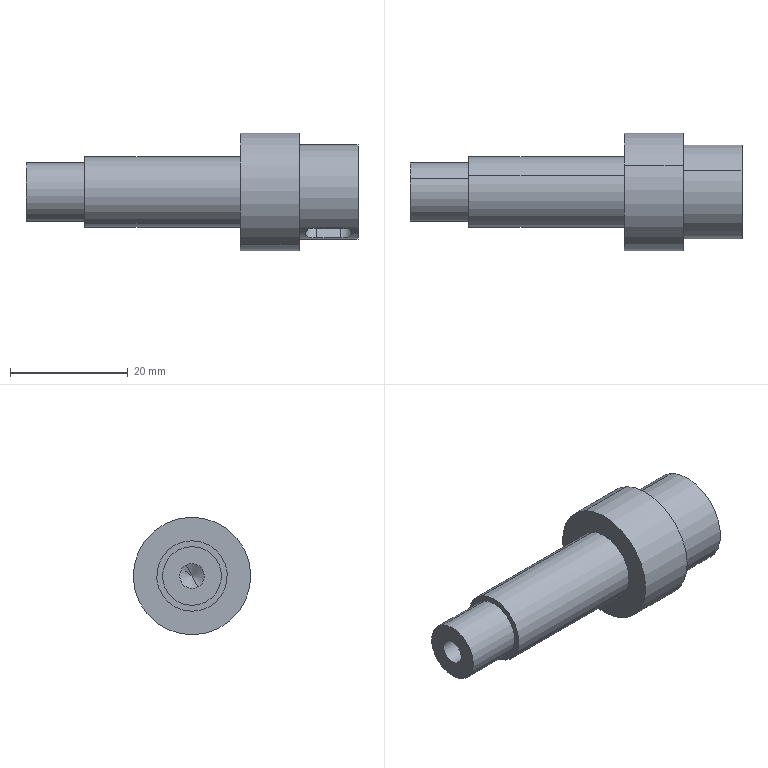Component | SolidWorks | ElectricalBoxAssembly2-1_SwingRodAxis-1 | 1 solid | 27 faces | box 56.5 x 20 x 20 mm | volume 8524 mm3 | cylinder 15 | plane 8 | cone 4 | commonest cylinder face diameters 4.2 x4 4 x3 16 x2 10 x2 12 x2 20 x2
build123d program:
from build123d import *

# Parameters (mm, degrees)
SKETCH1_R             = 10
BOSS_EXTRUDE1_DEPTH   = 10
SKETCH2_R             = 6
BOSS_EXTRUDE2_DEPTH   = 26.5
SKETCH3_R             = 5
BOSS_EXTRUDE3_DEPTH   = 10
M5_TAPPED_HOLE1_D     = 4.2
M5_TAPPED_HOLE1_DEPTH = 12.4
M5_TAPPED_HOLE1_TIP   = 1.262
SKETCH6_R             = 8
BOSS_EXTRUDE4_DEPTH   = 10
CUT_EXTRUDE1_DEPTH    = 2
M5_TAPPED_HOLE2_D     = 4.2
M5_TAPPED_HOLE2_DEPTH = 12.4
M5_TAPPED_HOLE2_TIP   = 1.262


with BuildPart() as part:
    # Sketch1 → Boss-Extrude1 (new body)
    with BuildSketch(Plane.XY):
        Circle(SKETCH1_R)
    extrude(amount=BOSS_EXTRUDE1_DEPTH)

    # Sketch2 → Boss-Extrude2 (add)
    with BuildSketch(Plane.XY.offset(10)):
        Circle(SKETCH2_R)
    extrude(amount=BOSS_EXTRUDE2_DEPTH)

    # Sketch3 → Boss-Extrude3 (add)
    with BuildSketch(Plane.XY.offset(36.5)):
        Circle(SKETCH3_R)
    extrude(amount=BOSS_EXTRUDE3_DEPTH)

    # M5 Tapped Hole1
    with Locations(Plane.XY.offset(46.5)):
        with Locations((0, 0)):
            Hole(M5_TAPPED_HOLE1_D / 2, depth=M5_TAPPED_HOLE1_DEPTH)
            with Locations((0, 0, -(M5_TAPPED_HOLE1_DEPTH + M5_TAPPED_HOLE1_TIP / 2))):  # 118° drill point
                Cone(0, M5_TAPPED_HOLE1_D / 2, M5_TAPPED_HOLE1_TIP, mode=Mode.SUBTRACT)

    # Sketch6 → Boss-Extrude4 (add)
    with BuildSketch(Plane(origin=(0, 0, 0), x_dir=(-1, 0, 0), z_dir=(0, 0, -1))):
        with Locations(Location((0, 0, 0), (0, 0, 180))):
            Circle(SKETCH6_R)
    extrude(amount=BOSS_EXTRUDE4_DEPTH)

    # Sketch7 → Cut-Extrude1 (cut)
    with BuildSketch(Plane(origin=(8, 0, 0), x_dir=(0, 0, -1), z_dir=(1, 0, 0))):
        with BuildLine():
            Line((3, 2), (7, 2))
            ThreePointArc((7, 2), (9, 0), (7, -2))
            Line((7, -2), (3, -2))
            ThreePointArc((3, -2), (1, 0), (3, 2))
        make_face()
    extrude(amount=-CUT_EXTRUDE1_DEPTH, mode=Mode.SUBTRACT)

    # M5 Tapped Hole2
    with Locations(Plane(origin=(0, 0, -10), x_dir=(-1, 0, 0), z_dir=(0, 0, -1))):
        with Locations((0, 0)):
            Hole(M5_TAPPED_HOLE2_D / 2, depth=M5_TAPPED_HOLE2_DEPTH)
            with Locations((0, 0, -(M5_TAPPED_HOLE2_DEPTH + M5_TAPPED_HOLE2_TIP / 2))):  # 118° drill point
                Cone(0, M5_TAPPED_HOLE2_D / 2, M5_TAPPED_HOLE2_TIP, mode=Mode.SUBTRACT)


solid = part.part

# Placed as in the assembly
solid = solid.moved(Location((786.968, 214.666, 1676.399), (152.899, -90, 0)))
STEP:
#1=COLOUR_RGB('',0.7922,0.8196,0.9333);
#2=FILL_AREA_STYLE_COLOUR('',#1);
#3=FILL_AREA_STYLE('',(#2));
#4=SURFACE_STYLE_FILL_AREA(#3);
#5=SURFACE_SIDE_STYLE('',(#4));
#6=SURFACE_STYLE_USAGE(.BOTH.,#5);
#7=PRESENTATION_STYLE_ASSIGNMENT((#6));
#8=CARTESIAN_POINT('',(30.889,8.414,65.926));
#9=VERTEX_POINT('',#8);
#10=CARTESIAN_POINT('',(30.889,8.489,66.074));
#11=VERTEX_POINT('',#10);
#12=CARTESIAN_POINT('',(30.889,8.451,66.));
#13=DIRECTION('',(1.,0.,0.));
#14=DIRECTION('',(0.,0.4556,0.8902));
#15=AXIS2_PLACEMENT_3D('',#12,#13,#14);
#16=CIRCLE('',#15,0.08268);
#17=EDGE_CURVE('',#9,#11,#16,.T.);
#18=ORIENTED_EDGE('',*,*,#17,.F.);
#19=CARTESIAN_POINT('',(31.377,8.414,65.926));
#20=VERTEX_POINT('',#19);
#21=CARTESIAN_POINT('',(31.377,8.414,65.926));
#22=DIRECTION('',(1.,0.,0.));
#23=VECTOR('',#22,39.37);
#24=LINE('',#21,#23);
#25=EDGE_CURVE('',#9,#20,#24,.T.);
#26=ORIENTED_EDGE('',*,*,#25,.T.);
#27=CARTESIAN_POINT('',(31.377,8.489,66.074));
#28=VERTEX_POINT('',#27);
#29=CARTESIAN_POINT('',(31.377,8.451,66.));
#30=DIRECTION('',(1.,0.,0.));
#31=DIRECTION('',(0.,0.4556,0.8902));
#32=AXIS2_PLACEMENT_3D('',#29,#30,#31);
#33=CIRCLE('',#32,0.08268);
#34=EDGE_CURVE('',#20,#28,#33,.T.);
#35=ORIENTED_EDGE('',*,*,#34,.T.);
#36=CARTESIAN_POINT('',(31.377,8.489,66.074));
#37=DIRECTION('',(1.,0.,0.));
#38=VECTOR('',#37,39.37);
#39=LINE('',#36,#38);
#40=EDGE_CURVE('',#11,#28,#39,.T.);
#41=ORIENTED_EDGE('',*,*,#40,.F.);
#42=EDGE_LOOP('',(#18,#26,#35,#41));
#43=FACE_OUTER_BOUND('',#42,.T.);
#44=CARTESIAN_POINT('',(31.377,8.451,66.));
#45=DIRECTION('',(1.,0.,0.));
#46=DIRECTION('',(0.,0.4556,0.8902));
#47=AXIS2_PLACEMENT_3D('',#44,#45,#46);
#48=CYLINDRICAL_SURFACE('',#47,0.08268);
#49=ADVANCED_FACE('',(#43),#48,.F.);
#50=CARTESIAN_POINT('',(30.839,8.451,66.));
#51=VERTEX_POINT('',#50);
#52=CARTESIAN_POINT('',(30.889,8.489,66.074));
#53=DIRECTION('',(0.515,0.3905,0.7631));
#54=VECTOR('',#53,39.37);
#55=LINE('',#52,#54);
#56=EDGE_CURVE('',#51,#11,#55,.T.);
#57=ORIENTED_EDGE('',*,*,#56,.F.);
#58=CARTESIAN_POINT('',(30.889,8.414,65.926));
#59=DIRECTION('',(0.515,-0.3905,-0.7631));
#60=VECTOR('',#59,39.37);
#61=LINE('',#58,#60);
#62=EDGE_CURVE('',#51,#9,#61,.T.);
#63=ORIENTED_EDGE('',*,*,#62,.T.);
#64=ORIENTED_EDGE('',*,*,#17,.T.);
#65=EDGE_LOOP('',(#57,#63,#64));
#66=FACE_OUTER_BOUND('',#65,.T.);
#67=CARTESIAN_POINT('',(30.889,8.451,66.));
#68=DIRECTION('',(1.,0.,0.));
#69=DIRECTION('',(0.,0.4556,0.8902));
#70=AXIS2_PLACEMENT_3D('',#67,#68,#69);
#71=CONICAL_SURFACE('',#70,0.08268,1.03);
#72=ADVANCED_FACE('',(#66),#71,.F.);
#73=CARTESIAN_POINT('',(31.337,8.344,65.79));
#74=VERTEX_POINT('',#73);
#75=CARTESIAN_POINT('',(31.259,8.274,65.826));
#76=VERTEX_POINT('',#75);
#77=CARTESIAN_POINT('',(31.259,8.344,65.79));
#78=DIRECTION('',(0.,-0.4556,-0.8902));
#79=DIRECTION('',(1.,0.,0.));
#80=AXIS2_PLACEMENT_3D('',#77,#78,#79);
#81=CIRCLE('',#80,0.07874);
#82=EDGE_CURVE('',#74,#76,#81,.T.);
#83=ORIENTED_EDGE('',*,*,#82,.F.);
#84=CARTESIAN_POINT('',(31.337,8.308,65.72));
#85=VERTEX_POINT('',#84);
#86=CARTESIAN_POINT('',(31.337,8.344,65.79));
#87=DIRECTION('',(0.,-0.4556,-0.8902));
#88=VECTOR('',#87,39.37);
#89=LINE('',#86,#88);
#90=EDGE_CURVE('',#74,#85,#89,.T.);
#91=ORIENTED_EDGE('',*,*,#90,.T.);
#92=CARTESIAN_POINT('',(31.259,8.242,65.764));
#93=VERTEX_POINT('',#92);
#94=CARTESIAN_POINT('',(31.259,8.242,65.764));
#95=CARTESIAN_POINT('',(31.264,8.242,65.764));
#96=CARTESIAN_POINT('',(31.269,8.243,65.764));
#97=CARTESIAN_POINT('',(31.279,8.244,65.763));
#98=CARTESIAN_POINT('',(31.284,8.246,65.762));
#99=CARTESIAN_POINT('',(31.294,8.249,65.759));
#100=CARTESIAN_POINT('',(31.298,8.251,65.757));
#101=CARTESIAN_POINT('',(31.307,8.255,65.754));
#102=CARTESIAN_POINT('',(31.311,8.258,65.752));
#103=CARTESIAN_POINT('',(31.322,8.266,65.745));
#104=CARTESIAN_POINT('',(31.327,8.274,65.74));
#105=CARTESIAN_POINT('',(31.333,8.286,65.732));
#106=CARTESIAN_POINT('',(31.335,8.29,65.729));
#107=CARTESIAN_POINT('',(31.337,8.299,65.724));
#108=CARTESIAN_POINT('',(31.337,8.303,65.722));
#109=CARTESIAN_POINT('',(31.337,8.308,65.72));
#110=B_SPLINE_CURVE_WITH_KNOTS('',3,(#94,#95,#96,#97,#98,#99,#100,#101,#102,#103,#104,#105,#106,#107,#108,#109),.UNSPECIFIED.,.F.,.F.,(4,2,2,2,2,2,2,4),(0.,0.0003925,0.0007849,0.001177,0.00157,0.002355,0.002747,0.00314),.UNSPECIFIED.);
#111=EDGE_CURVE('',#93,#85,#110,.T.);
#112=ORIENTED_EDGE('',*,*,#111,.F.);
#113=CARTESIAN_POINT('',(31.259,8.274,65.826));
#114=DIRECTION('',(0.,-0.4556,-0.8902));
#115=VECTOR('',#114,39.37);
#116=LINE('',#113,#115);
#117=EDGE_CURVE('',#76,#93,#116,.T.);
#118=ORIENTED_EDGE('',*,*,#117,.F.);
#119=EDGE_LOOP('',(#83,#91,#112,#118));
#120=FACE_OUTER_BOUND('',#119,.T.);
#121=CARTESIAN_POINT('',(31.259,8.344,65.79));
#122=DIRECTION('',(0.,-0.4556,-0.8902));
#123=DIRECTION('',(1.,0.,0.));
#124=AXIS2_PLACEMENT_3D('',#121,#122,#123);
#125=CYLINDRICAL_SURFACE('',#124,0.07874);
#126=ADVANCED_FACE('',(#120),#125,.F.);
#127=CARTESIAN_POINT('',(31.377,8.595,66.28));
#128=VERTEX_POINT('',#127);
#129=CARTESIAN_POINT('',(31.377,8.308,65.72));
#130=VERTEX_POINT('',#129);
#131=CARTESIAN_POINT('',(31.377,8.451,66.));
#132=DIRECTION('',(1.,0.,0.));
#133=DIRECTION('',(0.,0.4556,0.8902));
#134=AXIS2_PLACEMENT_3D('',#131,#132,#133);
#135=CIRCLE('',#134,0.315);
#136=EDGE_CURVE('',#128,#130,#135,.T.);
#137=ORIENTED_EDGE('',*,*,#136,.F.);
#138=CARTESIAN_POINT('',(30.983,8.595,66.28));
#139=VERTEX_POINT('',#138);
#140=CARTESIAN_POINT('',(31.377,8.595,66.28));
#141=DIRECTION('',(-1.,-0.,-0.));
#142=VECTOR('',#141,39.37);
#143=LINE('',#140,#142);
#144=EDGE_CURVE('',#128,#139,#143,.T.);
#145=ORIENTED_EDGE('',*,*,#144,.T.);
#146=CARTESIAN_POINT('',(30.983,8.308,65.72));
#147=VERTEX_POINT('',#146);
#148=CARTESIAN_POINT('',(30.983,8.451,66.));
#149=DIRECTION('',(1.,0.,0.));
#150=DIRECTION('',(0.,-0.4556,-0.8902));
#151=AXIS2_PLACEMENT_3D('',#148,#149,#150);
#152=CIRCLE('',#151,0.315);
#153=EDGE_CURVE('',#139,#147,#152,.T.);
#154=ORIENTED_EDGE('',*,*,#153,.T.);
#155=CARTESIAN_POINT('',(31.022,8.308,65.72));
#156=VERTEX_POINT('',#155);
#157=CARTESIAN_POINT('',(31.377,8.308,65.72));
#158=DIRECTION('',(-1.,-0.,-0.));
#159=VECTOR('',#158,39.37);
#160=LINE('',#157,#159);
#161=EDGE_CURVE('',#156,#147,#160,.T.);
#162=ORIENTED_EDGE('',*,*,#161,.F.);
#163=CARTESIAN_POINT('',(31.101,8.242,65.764));
#164=VERTEX_POINT('',#163);
#165=CARTESIAN_POINT('',(31.022,8.308,65.72));
#166=CARTESIAN_POINT('',(31.022,8.303,65.722));
#167=CARTESIAN_POINT('',(31.023,8.299,65.724));
#168=CARTESIAN_POINT('',(31.025,8.29,65.729));
#169=CARTESIAN_POINT('',(31.026,8.286,65.732));
#170=CARTESIAN_POINT('',(31.032,8.274,65.74));
#171=CARTESIAN_POINT('',(31.038,8.267,65.745));
#172=CARTESIAN_POINT('',(31.049,8.258,65.752));
#173=CARTESIAN_POINT('',(31.053,8.255,65.754));
#174=CARTESIAN_POINT('',(31.062,8.251,65.757));
#175=CARTESIAN_POINT('',(31.066,8.249,65.759));
#176=CARTESIAN_POINT('',(31.076,8.246,65.762));
#177=CARTESIAN_POINT('',(31.081,8.244,65.763));
#178=CARTESIAN_POINT('',(31.091,8.243,65.764));
#179=CARTESIAN_POINT('',(31.096,8.242,65.764));
#180=CARTESIAN_POINT('',(31.101,8.242,65.764));
#181=B_SPLINE_CURVE_WITH_KNOTS('',3,(#165,#166,#167,#168,#169,#170,#171,#172,#173,#174,#175,#176,#177,#178,#179,#180),.UNSPECIFIED.,.F.,.F.,(4,2,2,2,2,2,2,4),(0.00314,0.003532,0.003924,0.004708,0.0051,0.005492,0.005884,0.006276),.UNSPECIFIED.);
#182=EDGE_CURVE('',#156,#164,#181,.T.);
#183=ORIENTED_EDGE('',*,*,#182,.T.);
#184=CARTESIAN_POINT('',(31.377,8.242,65.764));
#185=DIRECTION('',(1.,0.,0.));
#186=VECTOR('',#185,39.37);
#187=LINE('',#184,#186);
#188=EDGE_CURVE('',#164,#93,#187,.T.);
#189=ORIENTED_EDGE('',*,*,#188,.T.);
#190=ORIENTED_EDGE('',*,*,#111,.T.);
#191=CARTESIAN_POINT('',(31.377,8.308,65.72));
#192=DIRECTION('',(-1.,-0.,-0.));
#193=VECTOR('',#192,39.37);
#194=LINE('',#191,#193);
#195=EDGE_CURVE('',#130,#85,#194,.T.);
#196=ORIENTED_EDGE('',*,*,#195,.F.);
#197=EDGE_LOOP('',(#137,#145,#154,#162,#183,#189,#190,#196));
#198=FACE_OUTER_BOUND('',#197,.T.);
#199=CARTESIAN_POINT('',(31.377,8.451,66.));
#200=DIRECTION('',(-1.,-0.,-0.));
#201=DIRECTION('',(0.,-0.4556,-0.8902));
#202=AXIS2_PLACEMENT_3D('',#199,#200,#201);
#203=CYLINDRICAL_SURFACE('',#202,0.315);
#204=ADVANCED_FACE('',(#198),#203,.T.);
#205=CARTESIAN_POINT('',(29.64,8.489,66.074));
#206=VERTEX_POINT('',#205);
#207=CARTESIAN_POINT('',(29.64,8.414,65.926));
#208=VERTEX_POINT('',#207);
#209=CARTESIAN_POINT('',(29.64,8.451,66.));
#210=DIRECTION('',(-1.,-0.,-0.));
#211=DIRECTION('',(0.,-0.4556,-0.8902));
#212=AXIS2_PLACEMENT_3D('',#209,#210,#211);
#213=CIRCLE('',#212,0.08268);
#214=EDGE_CURVE('',#206,#208,#213,.T.);
#215=ORIENTED_EDGE('',*,*,#214,.F.);
#216=CARTESIAN_POINT('',(29.152,8.489,66.074));
#217=VERTEX_POINT('',#216);
#218=CARTESIAN_POINT('',(29.152,8.489,66.074));
#219=DIRECTION('',(-1.,-0.,-0.));
#220=VECTOR('',#219,39.37);
#221=LINE('',#218,#220);
#222=EDGE_CURVE('',#206,#217,#221,.T.);
#223=ORIENTED_EDGE('',*,*,#222,.T.);
#224=CARTESIAN_POINT('',(29.152,8.414,65.926));
#225=VERTEX_POINT('',#224);
#226=CARTESIAN_POINT('',(29.152,8.451,66.));
#227=DIRECTION('',(-1.,-0.,-0.));
#228=DIRECTION('',(0.,-0.4556,-0.8902));
#229=AXIS2_PLACEMENT_3D('',#226,#227,#228);
#230=CIRCLE('',#229,0.08268);
#231=EDGE_CURVE('',#217,#225,#230,.T.);
#232=ORIENTED_EDGE('',*,*,#231,.T.);
#233=CARTESIAN_POINT('',(29.152,8.414,65.926));
#234=DIRECTION('',(-1.,-0.,-0.));
#235=VECTOR('',#234,39.37);
#236=LINE('',#233,#235);
#237=EDGE_CURVE('',#208,#225,#236,.T.);
#238=ORIENTED_EDGE('',*,*,#237,.F.);
#239=EDGE_LOOP('',(#215,#223,#232,#238));
#240=FACE_OUTER_BOUND('',#239,.T.);
#241=CARTESIAN_POINT('',(29.152,8.451,66.));
#242=DIRECTION('',(-1.,-0.,-0.));
#243=DIRECTION('',(0.,-0.4556,-0.8902));
#244=AXIS2_PLACEMENT_3D('',#241,#242,#243);
#245=CYLINDRICAL_SURFACE('',#244,0.08268);
#246=ADVANCED_FACE('',(#240),#245,.F.);
#247=CARTESIAN_POINT('',(29.69,8.451,66.));
#248=VERTEX_POINT('',#247);
#249=CARTESIAN_POINT('',(29.64,8.414,65.926));
#250=DIRECTION('',(-0.515,-0.3905,-0.7631));
#251=VECTOR('',#250,39.37);
#252=LINE('',#249,#251);
#253=EDGE_CURVE('',#248,#208,#252,.T.);
#254=ORIENTED_EDGE('',*,*,#253,.F.);
#255=CARTESIAN_POINT('',(29.64,8.489,66.074));
#256=DIRECTION('',(-0.515,0.3905,0.7631));
#257=VECTOR('',#256,39.37);
#258=LINE('',#255,#257);
#259=EDGE_CURVE('',#248,#206,#258,.T.);
#260=ORIENTED_EDGE('',*,*,#259,.T.);
#261=ORIENTED_EDGE('',*,*,#214,.T.);
#262=EDGE_LOOP('',(#254,#260,#261));
#263=FACE_OUTER_BOUND('',#262,.T.);
#264=CARTESIAN_POINT('',(29.64,8.451,66.));
#265=DIRECTION('',(-1.,-0.,-0.));
#266=DIRECTION('',(0.,-0.4556,-0.8902));
#267=AXIS2_PLACEMENT_3D('',#264,#265,#266);
#268=CONICAL_SURFACE('',#267,0.08268,1.03);
#269=ADVANCED_FACE('',(#263),#268,.F.);
#270=CARTESIAN_POINT('',(29.152,8.362,65.825));
#271=VERTEX_POINT('',#270);
#272=CARTESIAN_POINT('',(29.152,8.541,66.175));
#273=VERTEX_POINT('',#272);
#274=CARTESIAN_POINT('',(29.152,8.451,66.));
#275=DIRECTION('',(-1.,-0.,-0.));
#276=DIRECTION('',(0.,-0.4556,-0.8902));
#277=AXIS2_PLACEMENT_3D('',#274,#275,#276);
#278=CIRCLE('',#277,0.1969);
#279=EDGE_CURVE('',#271,#273,#278,.T.);
#280=ORIENTED_EDGE('',*,*,#279,.F.);
#281=CARTESIAN_POINT('',(29.546,8.362,65.825));
#282=VERTEX_POINT('',#281);
#283=CARTESIAN_POINT('',(29.152,8.362,65.825));
#284=DIRECTION('',(1.,0.,0.));
#285=VECTOR('',#284,39.37);
#286=LINE('',#283,#285);
#287=EDGE_CURVE('',#271,#282,#286,.T.);
#288=ORIENTED_EDGE('',*,*,#287,.T.);
#289=CARTESIAN_POINT('',(29.546,8.541,66.175));
#290=VERTEX_POINT('',#289);
#291=CARTESIAN_POINT('',(29.546,8.451,66.));
#292=DIRECTION('',(-1.,-0.,-0.));
#293=DIRECTION('',(0.,-0.4556,-0.8902));
#294=AXIS2_PLACEMENT_3D('',#291,#292,#293);
#295=CIRCLE('',#294,0.1969);
#296=EDGE_CURVE('',#282,#290,#295,.T.);
#297=ORIENTED_EDGE('',*,*,#296,.T.);
#298=CARTESIAN_POINT('',(29.152,8.541,66.175));
#299=DIRECTION('',(1.,0.,0.));
#300=VECTOR('',#299,39.37);
#301=LINE('',#298,#300);
#302=EDGE_CURVE('',#273,#290,#301,.T.);
#303=ORIENTED_EDGE('',*,*,#302,.F.);
#304=EDGE_LOOP('',(#280,#288,#297,#303));
#305=FACE_OUTER_BOUND('',#304,.T.);
#306=CARTESIAN_POINT('',(29.152,8.451,66.));
#307=DIRECTION('',(1.,0.,0.));
#308=DIRECTION('',(0.,0.4556,0.8902));
#309=AXIS2_PLACEMENT_3D('',#306,#307,#308);
#310=CYLINDRICAL_SURFACE('',#309,0.1969);
#311=ADVANCED_FACE('',(#305),#310,.T.);
#312=CARTESIAN_POINT('',(29.546,8.344,65.79));
#313=VERTEX_POINT('',#312);
#314=CARTESIAN_POINT('',(29.546,8.559,66.21));
#315=VERTEX_POINT('',#314);
#316=CARTESIAN_POINT('',(29.546,8.451,66.));
#317=DIRECTION('',(-1.,-0.,-0.));
#318=DIRECTION('',(0.,-0.4556,-0.8902));
#319=AXIS2_PLACEMENT_3D('',#316,#317,#318);
#320=CIRCLE('',#319,0.2362);
#321=EDGE_CURVE('',#313,#315,#320,.T.);
#322=ORIENTED_EDGE('',*,*,#321,.F.);
#323=CARTESIAN_POINT('',(30.589,8.344,65.79));
#324=VERTEX_POINT('',#323);
#325=CARTESIAN_POINT('',(29.546,8.344,65.79));
#326=DIRECTION('',(1.,0.,0.));
#327=VECTOR('',#326,39.37);
#328=LINE('',#325,#327);
#329=EDGE_CURVE('',#313,#324,#328,.T.);
#330=ORIENTED_EDGE('',*,*,#329,.T.);
#331=CARTESIAN_POINT('',(30.589,8.559,66.21));
#332=VERTEX_POINT('',#331);
#333=CARTESIAN_POINT('',(30.589,8.451,66.));
#334=DIRECTION('',(-1.,-0.,-0.));
#335=DIRECTION('',(0.,-0.4556,-0.8902));
#336=AXIS2_PLACEMENT_3D('',#333,#334,#335);
#337=CIRCLE('',#336,0.2362);
#338=EDGE_CURVE('',#324,#332,#337,.T.);
#339=ORIENTED_EDGE('',*,*,#338,.T.);
#340=CARTESIAN_POINT('',(29.546,8.559,66.21));
#341=DIRECTION('',(1.,0.,0.));
#342=VECTOR('',#341,39.37);
#343=LINE('',#340,#342);
#344=EDGE_CURVE('',#315,#332,#343,.T.);
#345=ORIENTED_EDGE('',*,*,#344,.F.);
#346=EDGE_LOOP('',(#322,#330,#339,#345));
#347=FACE_OUTER_BOUND('',#346,.T.);
#348=CARTESIAN_POINT('',(29.546,8.451,66.));
#349=DIRECTION('',(1.,0.,0.));
#350=DIRECTION('',(0.,0.4556,0.8902));
#351=AXIS2_PLACEMENT_3D('',#348,#349,#350);
#352=CYLINDRICAL_SURFACE('',#351,0.2362);
#353=ADVANCED_FACE('',(#347),#352,.T.);
#354=CARTESIAN_POINT('',(30.589,8.272,65.649));
#355=VERTEX_POINT('',#354);
#356=CARTESIAN_POINT('',(30.589,8.631,66.35));
#357=VERTEX_POINT('',#356);
#358=CARTESIAN_POINT('',(30.589,8.451,66.));
#359=DIRECTION('',(-1.,-0.,-0.));
#360=DIRECTION('',(0.,-0.4556,-0.8902));
#361=AXIS2_PLACEMENT_3D('',#358,#359,#360);
#362=CIRCLE('',#361,0.3937);
#363=EDGE_CURVE('',#355,#357,#362,.T.);
#364=ORIENTED_EDGE('',*,*,#363,.F.);
#365=CARTESIAN_POINT('',(30.983,8.272,65.649));
#366=VERTEX_POINT('',#365);
#367=CARTESIAN_POINT('',(30.589,8.272,65.649));
#368=DIRECTION('',(1.,0.,0.));
#369=VECTOR('',#368,39.37);
#370=LINE('',#367,#369);
#371=EDGE_CURVE('',#355,#366,#370,.T.);
#372=ORIENTED_EDGE('',*,*,#371,.T.);
#373=CARTESIAN_POINT('',(30.983,8.631,66.35));
#374=VERTEX_POINT('',#373);
#375=CARTESIAN_POINT('',(30.983,8.451,66.));
#376=DIRECTION('',(-1.,-0.,-0.));
#377=DIRECTION('',(0.,-0.4556,-0.8902));
#378=AXIS2_PLACEMENT_3D('',#375,#376,#377);
#379=CIRCLE('',#378,0.3937);
#380=EDGE_CURVE('',#366,#374,#379,.T.);
#381=ORIENTED_EDGE('',*,*,#380,.T.);
#382=CARTESIAN_POINT('',(30.589,8.631,66.35));
#383=DIRECTION('',(1.,0.,0.));
#384=VECTOR('',#383,39.37);
#385=LINE('',#382,#384);
#386=EDGE_CURVE('',#357,#374,#385,.T.);
#387=ORIENTED_EDGE('',*,*,#386,.F.);
#388=EDGE_LOOP('',(#364,#372,#381,#387));
#389=FACE_OUTER_BOUND('',#388,.T.);
#390=CARTESIAN_POINT('',(30.589,8.451,66.));
#391=DIRECTION('',(1.,0.,0.));
#392=DIRECTION('',(0.,0.4556,0.8902));
#393=AXIS2_PLACEMENT_3D('',#390,#391,#392);
#394=CYLINDRICAL_SURFACE('',#393,0.3937);
#395=ADVANCED_FACE('',(#389),#394,.T.);
#396=ORIENTED_EDGE('',*,*,#371,.F.);
#397=CARTESIAN_POINT('',(30.589,8.451,66.));
#398=DIRECTION('',(-1.,-0.,-0.));
#399=DIRECTION('',(0.,-0.4556,-0.8902));
#400=AXIS2_PLACEMENT_3D('',#397,#398,#399);
#401=CIRCLE('',#400,0.3937);
#402=EDGE_CURVE('',#357,#355,#401,.T.);
#403=ORIENTED_EDGE('',*,*,#402,.F.);
#404=ORIENTED_EDGE('',*,*,#386,.T.);
#405=CARTESIAN_POINT('',(30.983,8.451,66.));
#406=DIRECTION('',(-1.,-0.,-0.));
#407=DIRECTION('',(0.,-0.4556,-0.8902));
#408=AXIS2_PLACEMENT_3D('',#405,#406,#407);
#409=CIRCLE('',#408,0.3937);
#410=EDGE_CURVE('',#374,#366,#409,.T.);
#411=ORIENTED_EDGE('',*,*,#410,.T.);
#412=EDGE_LOOP('',(#396,#403,#404,#411));
#413=FACE_OUTER_BOUND('',#412,.T.);
#414=CARTESIAN_POINT('',(30.589,8.451,66.));
#415=DIRECTION('',(1.,0.,0.));
#416=DIRECTION('',(0.,0.4556,0.8902));
#417=AXIS2_PLACEMENT_3D('',#414,#415,#416);
#418=CYLINDRICAL_SURFACE('',#417,0.3937);
#419=ADVANCED_FACE('',(#413),#418,.T.);
#420=CARTESIAN_POINT('',(30.589,8.451,66.));
#421=DIRECTION('',(-1.,-0.,-0.));
#422=DIRECTION('',(0.,-0.4556,-0.8902));
#423=AXIS2_PLACEMENT_3D('',#420,#421,#422);
#424=CIRCLE('',#423,0.2362);
#425=EDGE_CURVE('',#332,#324,#424,.T.);
#426=ORIENTED_EDGE('',*,*,#425,.F.);
#427=ORIENTED_EDGE('',*,*,#338,.F.);
#428=EDGE_LOOP('',(#426,#427));
#429=FACE_BOUND('',#428,.T.);
#430=ORIENTED_EDGE('',*,*,#402,.T.);
#431=ORIENTED_EDGE('',*,*,#363,.T.);
#432=EDGE_LOOP('',(#430,#431));
#433=FACE_OUTER_BOUND('',#432,.T.);
#434=CARTESIAN_POINT('',(30.589,8.451,66.));
#435=DIRECTION('',(-1.,-0.,-0.));
#436=DIRECTION('',(0.,-0.4556,-0.8902));
#437=AXIS2_PLACEMENT_3D('',#434,#435,#436);
#438=PLANE('',#437);
#439=ADVANCED_FACE('',(#429,#433),#438,.T.);
#440=CARTESIAN_POINT('',(30.983,8.451,66.));
#441=DIRECTION('',(1.,0.,0.));
#442=DIRECTION('',(0.,-0.4556,-0.8902));
#443=AXIS2_PLACEMENT_3D('',#440,#441,#442);
#444=CIRCLE('',#443,0.315);
#445=EDGE_CURVE('',#147,#139,#444,.T.);
#446=ORIENTED_EDGE('',*,*,#445,.F.);
#447=ORIENTED_EDGE('',*,*,#153,.F.);
#448=EDGE_LOOP('',(#446,#447));
#449=FACE_BOUND('',#448,.T.);
#450=ORIENTED_EDGE('',*,*,#410,.F.);
#451=ORIENTED_EDGE('',*,*,#380,.F.);
#452=EDGE_LOOP('',(#450,#451));
#453=FACE_OUTER_BOUND('',#452,.T.);
#454=CARTESIAN_POINT('',(30.983,8.451,66.));
#455=DIRECTION('',(-1.,-0.,-0.));
#456=DIRECTION('',(0.,-0.4556,-0.8902));
#457=AXIS2_PLACEMENT_3D('',#454,#455,#456);
#458=PLANE('',#457);
#459=ADVANCED_FACE('',(#449,#453),#458,.F.);
#460=ORIENTED_EDGE('',*,*,#329,.F.);
#461=CARTESIAN_POINT('',(29.546,8.451,66.));
#462=DIRECTION('',(-1.,-0.,-0.));
#463=DIRECTION('',(0.,-0.4556,-0.8902));
#464=AXIS2_PLACEMENT_3D('',#461,#462,#463);
#465=CIRCLE('',#464,0.2362);
#466=EDGE_CURVE('',#315,#313,#465,.T.);
#467=ORIENTED_EDGE('',*,*,#466,.F.);
#468=ORIENTED_EDGE('',*,*,#344,.T.);
#469=ORIENTED_EDGE('',*,*,#425,.T.);
#470=EDGE_LOOP('',(#460,#467,#468,#469));
#471=FACE_OUTER_BOUND('',#470,.T.);
#472=CARTESIAN_POINT('',(29.546,8.451,66.));
#473=DIRECTION('',(1.,0.,0.));
#474=DIRECTION('',(0.,0.4556,0.8902));
#475=AXIS2_PLACEMENT_3D('',#472,#473,#474);
#476=CYLINDRICAL_SURFACE('',#475,0.2362);
#477=ADVANCED_FACE('',(#471),#476,.T.);
#478=CARTESIAN_POINT('',(29.546,8.451,66.));
#479=DIRECTION('',(-1.,-0.,-0.));
#480=DIRECTION('',(0.,-0.4556,-0.8902));
#481=AXIS2_PLACEMENT_3D('',#478,#479,#480);
#482=CIRCLE('',#481,0.1969);
#483=EDGE_CURVE('',#290,#282,#482,.T.);
#484=ORIENTED_EDGE('',*,*,#483,.F.);
#485=ORIENTED_EDGE('',*,*,#296,.F.);
#486=EDGE_LOOP('',(#484,#485));
#487=FACE_BOUND('',#486,.T.);
#488=ORIENTED_EDGE('',*,*,#466,.T.);
#489=ORIENTED_EDGE('',*,*,#321,.T.);
#490=EDGE_LOOP('',(#488,#489));
#491=FACE_OUTER_BOUND('',#490,.T.);
#492=CARTESIAN_POINT('',(29.546,8.451,66.));
#493=DIRECTION('',(-1.,-0.,-0.));
#494=DIRECTION('',(0.,-0.4556,-0.8902));
#495=AXIS2_PLACEMENT_3D('',#492,#493,#494);
#496=PLANE('',#495);
#497=ADVANCED_FACE('',(#487,#491),#496,.T.);
#498=ORIENTED_EDGE('',*,*,#287,.F.);
#499=CARTESIAN_POINT('',(29.152,8.451,66.));
#500=DIRECTION('',(-1.,-0.,-0.));
#501=DIRECTION('',(0.,-0.4556,-0.8902));
#502=AXIS2_PLACEMENT_3D('',#499,#500,#501);
#503=CIRCLE('',#502,0.1969);
#504=EDGE_CURVE('',#273,#271,#503,.T.);
#505=ORIENTED_EDGE('',*,*,#504,.F.);
#506=ORIENTED_EDGE('',*,*,#302,.T.);
#507=ORIENTED_EDGE('',*,*,#483,.T.);
#508=EDGE_LOOP('',(#498,#505,#506,#507));
#509=FACE_OUTER_BOUND('',#508,.T.);
#510=CARTESIAN_POINT('',(29.152,8.451,66.));
#511=DIRECTION('',(1.,0.,0.));
#512=DIRECTION('',(0.,0.4556,0.8902));
#513=AXIS2_PLACEMENT_3D('',#510,#511,#512);
#514=CYLINDRICAL_SURFACE('',#513,0.1969);
#515=ADVANCED_FACE('',(#509),#514,.T.);
#516=CARTESIAN_POINT('',(29.152,8.451,66.));
#517=DIRECTION('',(-1.,-0.,-0.));
#518=DIRECTION('',(0.,-0.4556,-0.8902));
#519=AXIS2_PLACEMENT_3D('',#516,#517,#518);
#520=CIRCLE('',#519,0.08268);
#521=EDGE_CURVE('',#225,#217,#520,.T.);
#522=ORIENTED_EDGE('',*,*,#521,.F.);
#523=ORIENTED_EDGE('',*,*,#231,.F.);
#524=EDGE_LOOP('',(#522,#523));
#525=FACE_BOUND('',#524,.T.);
#526=ORIENTED_EDGE('',*,*,#504,.T.);
#527=ORIENTED_EDGE('',*,*,#279,.T.);
#528=EDGE_LOOP('',(#526,#527));
#529=FACE_OUTER_BOUND('',#528,.T.);
#530=CARTESIAN_POINT('',(29.152,8.451,66.));
#531=DIRECTION('',(-1.,-0.,-0.));
#532=DIRECTION('',(0.,-0.4556,-0.8902));
#533=AXIS2_PLACEMENT_3D('',#530,#531,#532);
#534=PLANE('',#533);
#535=ADVANCED_FACE('',(#525,#529),#534,.T.);
#536=ORIENTED_EDGE('',*,*,#259,.F.);
#537=ORIENTED_EDGE('',*,*,#253,.T.);
#538=CARTESIAN_POINT('',(29.64,8.451,66.));
#539=DIRECTION('',(-1.,-0.,-0.));
#540=DIRECTION('',(0.,-0.4556,-0.8902));
#541=AXIS2_PLACEMENT_3D('',#538,#539,#540);
#542=CIRCLE('',#541,0.08268);
#543=EDGE_CURVE('',#208,#206,#542,.T.);
#544=ORIENTED_EDGE('',*,*,#543,.T.);
#545=EDGE_LOOP('',(#536,#537,#544));
#546=FACE_OUTER_BOUND('',#545,.T.);
#547=CARTESIAN_POINT('',(29.64,8.451,66.));
#548=DIRECTION('',(-1.,-0.,-0.));
#549=DIRECTION('',(0.,-0.4556,-0.8902));
#550=AXIS2_PLACEMENT_3D('',#547,#548,#549);
#551=CONICAL_SURFACE('',#550,0.08268,1.03);
#552=ADVANCED_FACE('',(#546),#551,.F.);
#553=ORIENTED_EDGE('',*,*,#222,.F.);
#554=ORIENTED_EDGE('',*,*,#543,.F.);
#555=ORIENTED_EDGE('',*,*,#237,.T.);
#556=ORIENTED_EDGE('',*,*,#521,.T.);
#557=EDGE_LOOP('',(#553,#554,#555,#556));
#558=FACE_OUTER_BOUND('',#557,.T.);
#559=CARTESIAN_POINT('',(29.152,8.451,66.));
#560=DIRECTION('',(-1.,-0.,-0.));
#561=DIRECTION('',(0.,-0.4556,-0.8902));
#562=AXIS2_PLACEMENT_3D('',#559,#560,#561);
#563=CYLINDRICAL_SURFACE('',#562,0.08268);
#564=ADVANCED_FACE('',(#558),#563,.F.);
#565=ORIENTED_EDGE('',*,*,#144,.F.);
#566=CARTESIAN_POINT('',(31.377,8.451,66.));
#567=DIRECTION('',(1.,0.,0.));
#568=DIRECTION('',(0.,0.4556,0.8902));
#569=AXIS2_PLACEMENT_3D('',#566,#567,#568);
#570=CIRCLE('',#569,0.315);
#571=EDGE_CURVE('',#130,#128,#570,.T.);
#572=ORIENTED_EDGE('',*,*,#571,.F.);
#573=ORIENTED_EDGE('',*,*,#195,.T.);
#574=CARTESIAN_POINT('',(31.259,8.383,65.693));
#575=VERTEX_POINT('',#574);
#576=CARTESIAN_POINT('',(31.337,8.308,65.72));
#577=CARTESIAN_POINT('',(31.337,8.313,65.717));
#578=CARTESIAN_POINT('',(31.337,8.317,65.715));
#579=CARTESIAN_POINT('',(31.335,8.326,65.711));
#580=CARTESIAN_POINT('',(31.333,8.331,65.709));
#581=CARTESIAN_POINT('',(31.327,8.344,65.704));
#582=CARTESIAN_POINT('',(31.322,8.353,65.701));
#583=CARTESIAN_POINT('',(31.311,8.363,65.698));
#584=CARTESIAN_POINT('',(31.307,8.366,65.697));
#585=CARTESIAN_POINT('',(31.298,8.372,65.695));
#586=CARTESIAN_POINT('',(31.294,8.375,65.695));
#587=CARTESIAN_POINT('',(31.284,8.379,65.694));
#588=CARTESIAN_POINT('',(31.279,8.38,65.693));
#589=CARTESIAN_POINT('',(31.269,8.382,65.693));
#590=CARTESIAN_POINT('',(31.264,8.383,65.693));
#591=CARTESIAN_POINT('',(31.259,8.383,65.693));
#592=B_SPLINE_CURVE_WITH_KNOTS('',3,(#576,#577,#578,#579,#580,#581,#582,#583,#584,#585,#586,#587,#588,#589,#590,#591),.UNSPECIFIED.,.F.,.F.,(4,2,2,2,2,2,2,4),(0.00314,0.003532,0.003924,0.004708,0.0051,0.005492,0.005884,0.006276),.UNSPECIFIED.);
#593=EDGE_CURVE('',#85,#575,#592,.T.);
#594=ORIENTED_EDGE('',*,*,#593,.T.);
#595=CARTESIAN_POINT('',(31.101,8.383,65.693));
#596=VERTEX_POINT('',#595);
#597=CARTESIAN_POINT('',(31.377,8.383,65.693));
#598=DIRECTION('',(-1.,-0.,-0.));
#599=VECTOR('',#598,39.37);
#600=LINE('',#597,#599);
#601=EDGE_CURVE('',#575,#596,#600,.T.);
#602=ORIENTED_EDGE('',*,*,#601,.T.);
#603=CARTESIAN_POINT('',(31.101,8.383,65.693));
#604=CARTESIAN_POINT('',(31.096,8.383,65.693));
#605=CARTESIAN_POINT('',(31.091,8.382,65.693));
#606=CARTESIAN_POINT('',(31.081,8.38,65.693));
#607=CARTESIAN_POINT('',(31.076,8.379,65.694));
#608=CARTESIAN_POINT('',(31.066,8.375,65.695));
#609=CARTESIAN_POINT('',(31.062,8.372,65.695));
#610=CARTESIAN_POINT('',(31.053,8.366,65.697));
#611=CARTESIAN_POINT('',(31.049,8.363,65.698));
#612=CARTESIAN_POINT('',(31.038,8.353,65.701));
#613=CARTESIAN_POINT('',(31.032,8.344,65.704));
#614=CARTESIAN_POINT('',(31.026,8.331,65.709));
#615=CARTESIAN_POINT('',(31.025,8.326,65.711));
#616=CARTESIAN_POINT('',(31.023,8.317,65.715));
#617=CARTESIAN_POINT('',(31.022,8.313,65.717));
#618=CARTESIAN_POINT('',(31.022,8.308,65.72));
#619=B_SPLINE_CURVE_WITH_KNOTS('',3,(#603,#604,#605,#606,#607,#608,#609,#610,#611,#612,#613,#614,#615,#616,#617,#618),.UNSPECIFIED.,.F.,.F.,(4,2,2,2,2,2,2,4),(0.,0.0003925,0.0007849,0.001177,0.00157,0.002355,0.002747,0.00314),.UNSPECIFIED.);
#620=EDGE_CURVE('',#596,#156,#619,.T.);
#621=ORIENTED_EDGE('',*,*,#620,.T.);
#622=ORIENTED_EDGE('',*,*,#161,.T.);
#623=ORIENTED_EDGE('',*,*,#445,.T.);
#624=EDGE_LOOP('',(#565,#572,#573,#594,#602,#621,#622,#623));
#625=FACE_OUTER_BOUND('',#624,.T.);
#626=CARTESIAN_POINT('',(31.377,8.451,66.));
#627=DIRECTION('',(-1.,-0.,-0.));
#628=DIRECTION('',(0.,-0.4556,-0.8902));
#629=AXIS2_PLACEMENT_3D('',#626,#627,#628);
#630=CYLINDRICAL_SURFACE('',#629,0.315);
#631=ADVANCED_FACE('',(#625),#630,.T.);
#632=CARTESIAN_POINT('',(31.377,8.451,66.));
#633=DIRECTION('',(1.,0.,0.));
#634=DIRECTION('',(0.,0.4556,0.8902));
#635=AXIS2_PLACEMENT_3D('',#632,#633,#634);
#636=CIRCLE('',#635,0.08268);
#637=EDGE_CURVE('',#28,#20,#636,.T.);
#638=ORIENTED_EDGE('',*,*,#637,.F.);
#639=ORIENTED_EDGE('',*,*,#34,.F.);
#640=EDGE_LOOP('',(#638,#639));
#641=FACE_BOUND('',#640,.T.);
#642=ORIENTED_EDGE('',*,*,#571,.T.);
#643=ORIENTED_EDGE('',*,*,#136,.T.);
#644=EDGE_LOOP('',(#642,#643));
#645=FACE_OUTER_BOUND('',#644,.T.);
#646=CARTESIAN_POINT('',(31.377,8.451,66.));
#647=DIRECTION('',(1.,0.,0.));
#648=DIRECTION('',(-0.,0.4556,0.8902));
#649=AXIS2_PLACEMENT_3D('',#646,#647,#648);
#650=PLANE('',#649);
#651=ADVANCED_FACE('',(#641,#645),#650,.T.);
#652=CARTESIAN_POINT('',(31.101,8.414,65.754));
#653=VERTEX_POINT('',#652);
#654=CARTESIAN_POINT('',(31.101,8.414,65.754));
#655=DIRECTION('',(0.,-0.4556,-0.8902));
#656=VECTOR('',#655,39.37);
#657=LINE('',#654,#656);
#658=EDGE_CURVE('',#653,#596,#657,.T.);
#659=ORIENTED_EDGE('',*,*,#658,.F.);
#660=CARTESIAN_POINT('',(31.101,8.274,65.826));
#661=VERTEX_POINT('',#660);
#662=CARTESIAN_POINT('',(31.101,8.344,65.79));
#663=DIRECTION('',(0.,-0.4556,-0.8902));
#664=DIRECTION('',(1.,0.,0.));
#665=AXIS2_PLACEMENT_3D('',#662,#663,#664);
#666=CIRCLE('',#665,0.07874);
#667=EDGE_CURVE('',#661,#653,#666,.T.);
#668=ORIENTED_EDGE('',*,*,#667,.F.);
#669=CARTESIAN_POINT('',(31.101,8.274,65.826));
#670=DIRECTION('',(0.,-0.4556,-0.8902));
#671=VECTOR('',#670,39.37);
#672=LINE('',#669,#671);
#673=EDGE_CURVE('',#661,#164,#672,.T.);
#674=ORIENTED_EDGE('',*,*,#673,.T.);
#675=ORIENTED_EDGE('',*,*,#182,.F.);
#676=ORIENTED_EDGE('',*,*,#620,.F.);
#677=EDGE_LOOP('',(#659,#668,#674,#675,#676));
#678=FACE_OUTER_BOUND('',#677,.T.);
#679=CARTESIAN_POINT('',(31.101,8.344,65.79));
#680=DIRECTION('',(0.,-0.4556,-0.8902));
#681=DIRECTION('',(1.,0.,0.));
#682=AXIS2_PLACEMENT_3D('',#679,#680,#681);
#683=CYLINDRICAL_SURFACE('',#682,0.07874);
#684=ADVANCED_FACE('',(#678),#683,.F.);
#685=ORIENTED_EDGE('',*,*,#673,.F.);
#686=CARTESIAN_POINT('',(31.101,8.274,65.826));
#687=DIRECTION('',(-1.,0.,-0.));
#688=VECTOR('',#687,39.37);
#689=LINE('',#686,#688);
#690=EDGE_CURVE('',#76,#661,#689,.T.);
#691=ORIENTED_EDGE('',*,*,#690,.F.);
#692=ORIENTED_EDGE('',*,*,#117,.T.);
#693=ORIENTED_EDGE('',*,*,#188,.F.);
#694=EDGE_LOOP('',(#685,#691,#692,#693));
#695=FACE_OUTER_BOUND('',#694,.T.);
#696=CARTESIAN_POINT('',(31.101,8.274,65.826));
#697=DIRECTION('',(-0.,-0.8902,0.4556));
#698=DIRECTION('',(-1.,0.,-0.));
#699=AXIS2_PLACEMENT_3D('',#696,#697,#698);
#700=PLANE('',#699);
#701=ADVANCED_FACE('',(#695),#700,.F.);
#702=ORIENTED_EDGE('',*,*,#90,.F.);
#703=CARTESIAN_POINT('',(31.259,8.414,65.754));
#704=VERTEX_POINT('',#703);
#705=CARTESIAN_POINT('',(31.259,8.344,65.79));
#706=DIRECTION('',(0.,-0.4556,-0.8902));
#707=DIRECTION('',(1.,0.,0.));
#708=AXIS2_PLACEMENT_3D('',#705,#706,#707);
#709=CIRCLE('',#708,0.07874);
#710=EDGE_CURVE('',#704,#74,#709,.T.);
#711=ORIENTED_EDGE('',*,*,#710,.F.);
#712=CARTESIAN_POINT('',(31.259,8.414,65.754));
#713=DIRECTION('',(0.,-0.4556,-0.8902));
#714=VECTOR('',#713,39.37);
#715=LINE('',#712,#714);
#716=EDGE_CURVE('',#704,#575,#715,.T.);
#717=ORIENTED_EDGE('',*,*,#716,.T.);
#718=ORIENTED_EDGE('',*,*,#593,.F.);
#719=EDGE_LOOP('',(#702,#711,#717,#718));
#720=FACE_OUTER_BOUND('',#719,.T.);
#721=CARTESIAN_POINT('',(31.259,8.344,65.79));
#722=DIRECTION('',(0.,-0.4556,-0.8902));
#723=DIRECTION('',(1.,0.,0.));
#724=AXIS2_PLACEMENT_3D('',#721,#722,#723);
#725=CYLINDRICAL_SURFACE('',#724,0.07874);
#726=ADVANCED_FACE('',(#720),#725,.F.);
#727=ORIENTED_EDGE('',*,*,#716,.F.);
#728=CARTESIAN_POINT('',(31.101,8.414,65.754));
#729=DIRECTION('',(1.,-0.,0.));
#730=VECTOR('',#729,39.37);
#731=LINE('',#728,#730);
#732=EDGE_CURVE('',#653,#704,#731,.T.);
#733=ORIENTED_EDGE('',*,*,#732,.F.);
#734=ORIENTED_EDGE('',*,*,#658,.T.);
#735=ORIENTED_EDGE('',*,*,#601,.F.);
#736=EDGE_LOOP('',(#727,#733,#734,#735));
#737=FACE_OUTER_BOUND('',#736,.T.);
#738=CARTESIAN_POINT('',(31.101,8.414,65.754));
#739=DIRECTION('',(0.,0.8902,-0.4556));
#740=DIRECTION('',(1.,-0.,0.));
#741=AXIS2_PLACEMENT_3D('',#738,#739,#740);
#742=PLANE('',#741);
#743=ADVANCED_FACE('',(#737),#742,.F.);
#744=ORIENTED_EDGE('',*,*,#667,.T.);
#745=ORIENTED_EDGE('',*,*,#732,.T.);
#746=ORIENTED_EDGE('',*,*,#710,.T.);
#747=ORIENTED_EDGE('',*,*,#82,.T.);
#748=ORIENTED_EDGE('',*,*,#690,.T.);
#749=EDGE_LOOP('',(#744,#745,#746,#747,#748));
#750=FACE_OUTER_BOUND('',#749,.T.);
#751=CARTESIAN_POINT('',(31.101,8.344,65.79));
#752=DIRECTION('',(0.,-0.4556,-0.8902));
#753=DIRECTION('',(1.,0.,0.));
#754=AXIS2_PLACEMENT_3D('',#751,#752,#753);
#755=PLANE('',#754);
#756=ADVANCED_FACE('',(#750),#755,.T.);
#757=ORIENTED_EDGE('',*,*,#62,.F.);
#758=ORIENTED_EDGE('',*,*,#56,.T.);
#759=CARTESIAN_POINT('',(30.889,8.451,66.));
#760=DIRECTION('',(1.,0.,0.));
#761=DIRECTION('',(0.,0.4556,0.8902));
#762=AXIS2_PLACEMENT_3D('',#759,#760,#761);
#763=CIRCLE('',#762,0.08268);
#764=EDGE_CURVE('',#11,#9,#763,.T.);
#765=ORIENTED_EDGE('',*,*,#764,.T.);
#766=EDGE_LOOP('',(#757,#758,#765));
#767=FACE_OUTER_BOUND('',#766,.T.);
#768=CARTESIAN_POINT('',(30.889,8.451,66.));
#769=DIRECTION('',(1.,0.,0.));
#770=DIRECTION('',(0.,0.4556,0.8902));
#771=AXIS2_PLACEMENT_3D('',#768,#769,#770);
#772=CONICAL_SURFACE('',#771,0.08268,1.03);
#773=ADVANCED_FACE('',(#767),#772,.F.);
#774=ORIENTED_EDGE('',*,*,#25,.F.);
#775=ORIENTED_EDGE('',*,*,#764,.F.);
#776=ORIENTED_EDGE('',*,*,#40,.T.);
#777=ORIENTED_EDGE('',*,*,#637,.T.);
#778=EDGE_LOOP('',(#774,#775,#776,#777));
#779=FACE_OUTER_BOUND('',#778,.T.);
#780=CARTESIAN_POINT('',(31.377,8.451,66.));
#781=DIRECTION('',(1.,0.,0.));
#782=DIRECTION('',(0.,0.4556,0.8902));
#783=AXIS2_PLACEMENT_3D('',#780,#781,#782);
#784=CYLINDRICAL_SURFACE('',#783,0.08268);
#785=ADVANCED_FACE('',(#779),#784,.F.);
#786=CLOSED_SHELL('',(#49,#72,#126,#204,#246,#269,#311,#353,#395,#419,#439,#459,#477,#497,#515,#535,#552,#564,#631,#651,#684,#701,#726,#743,#756,#773,#785));
#787=MANIFOLD_SOLID_BREP('',#786);
#788=STYLED_ITEM('',(#7),#787);
#789=(LENGTH_UNIT()NAMED_UNIT(*)SI_UNIT($,.METRE.));
#790=LENGTH_MEASURE_WITH_UNIT(LENGTH_MEASURE(0.0254),#789);
#791=DIMENSIONAL_EXPONENTS(1.,0.,0.,0.,0.,0.,0.);
#792=(CONVERSION_BASED_UNIT('',#790)LENGTH_UNIT()NAMED_UNIT(#791));
#793=UNCERTAINTY_MEASURE_WITH_UNIT(LENGTH_MEASURE(0.00001),#792,'','');
#794=(NAMED_UNIT(*)PLANE_ANGLE_UNIT()SI_UNIT($,.RADIAN.));
#795=(NAMED_UNIT(*)SI_UNIT($,.STERADIAN.)SOLID_ANGLE_UNIT());
#796=(GEOMETRIC_REPRESENTATION_CONTEXT(3)GLOBAL_UNCERTAINTY_ASSIGNED_CONTEXT((#793))GLOBAL_UNIT_ASSIGNED_CONTEXT((#792,#794,#795))REPRESENTATION_CONTEXT('',''));
#797=MECHANICAL_DESIGN_GEOMETRIC_PRESENTATION_REPRESENTATION('',(#788),#796);
#798=CARTESIAN_POINT('',(0.,0.,0.));
#799=DIRECTION('',(0.,0.,1.));
#800=DIRECTION('',(1.,0.,0.));
#801=AXIS2_PLACEMENT_3D('',#798,#799,#800);
#802=(LENGTH_UNIT()NAMED_UNIT(*)SI_UNIT($,.METRE.));
#803=LENGTH_MEASURE_WITH_UNIT(LENGTH_MEASURE(0.0254),#802);
#804=DIMENSIONAL_EXPONENTS(1.,0.,0.,0.,0.,0.,0.);
#805=(CONVERSION_BASED_UNIT('',#803)LENGTH_UNIT()NAMED_UNIT(#804));
#806=UNCERTAINTY_MEASURE_WITH_UNIT(LENGTH_MEASURE(0.00001),#805,'','');
#807=(NAMED_UNIT(*)PLANE_ANGLE_UNIT()SI_UNIT($,.RADIAN.));
#808=(NAMED_UNIT(*)SI_UNIT($,.STERADIAN.)SOLID_ANGLE_UNIT());
#809=(GEOMETRIC_REPRESENTATION_CONTEXT(3)GLOBAL_UNCERTAINTY_ASSIGNED_CONTEXT((#806))GLOBAL_UNIT_ASSIGNED_CONTEXT((#805,#807,#808))REPRESENTATION_CONTEXT('',''));
#810=ADVANCED_BREP_SHAPE_REPRESENTATION('',(#787,#801),#809);
#811=PRESENTATION_LAYER_ASSIGNMENT('','',(#788));